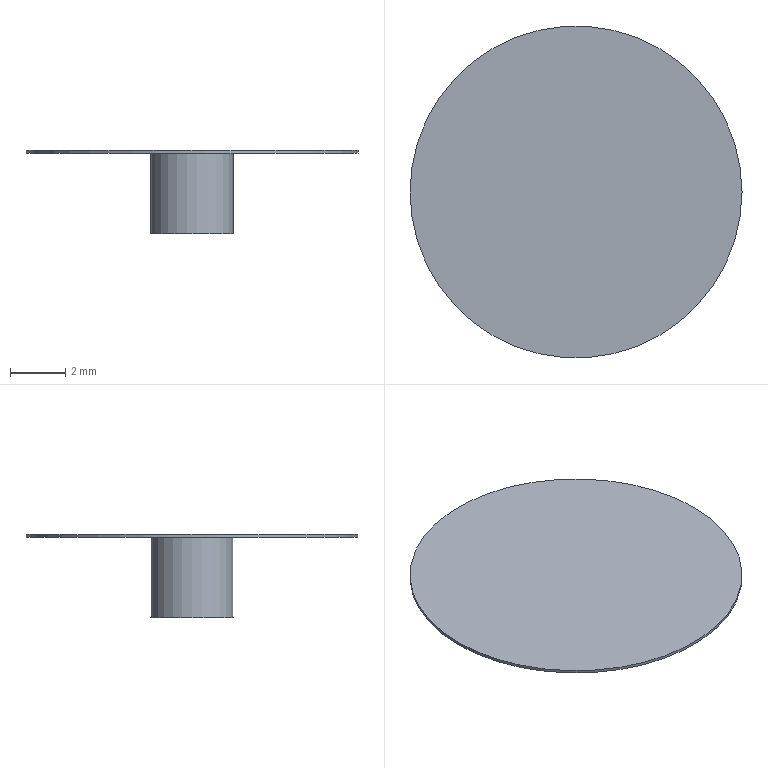Component | NX | ROBOT_ARM_FLANGE | 1 solid | 5 faces | box 12 x 12 x 3 mm | volume 32 mm3 | plane 3 | cylinder 2 | commonest cylinder face diameters 3 x1 12 x1
STEP:
#1=CARTESIAN_POINT('',(0.,0.,0.));
#2=DIRECTION('',(0.,0.,1.));
#3=DIRECTION('',(1.,0.,0.));
#4=AXIS2_PLACEMENT_3D('',#1,#2,#3);
#5=CARTESIAN_POINT('',(15.971,14.526,113.674));
#6=VERTEX_POINT('',#5);
#7=CARTESIAN_POINT('',(14.471,14.526,113.674));
#8=DIRECTION('',(0.,0.,1.));
#9=DIRECTION('',(1.,0.,0.));
#10=AXIS2_PLACEMENT_3D('',#7,#8,#9);
#11=CIRCLE('',#10,1.5);
#12=CARTESIAN_POINT('',(14.471,14.526,113.674));
#13=DIRECTION('',(0.,0.,1.));
#14=DIRECTION('',(1.,0.,0.));
#15=AXIS2_PLACEMENT_3D('',#12,#13,#14);
#16=CYLINDRICAL_SURFACE('',#15,1.5);
#17=CARTESIAN_POINT('',(0.,0.));
#18=DIRECTION('',(1.,0.));
#19=VECTOR('',#18,1.);
#20=LINE('',#17,#19);
#21=(GEOMETRIC_REPRESENTATION_CONTEXT(2)PARAMETRIC_REPRESENTATION_CONTEXT()REPRESENTATION_CONTEXT('',''));
#22=DEFINITIONAL_REPRESENTATION('',(#20),#21);
#23=PCURVE('',#16,#22);
#24=CARTESIAN_POINT('',(14.471,14.526,113.674));
#25=DIRECTION('',(0.,0.,1.));
#26=DIRECTION('',(1.,0.,0.));
#27=AXIS2_PLACEMENT_3D('',#24,#25,#26);
#28=PLANE('',#27);
#29=CARTESIAN_POINT('',(0.,0.));
#30=DIRECTION('',(1.,0.));
#31=AXIS2_PLACEMENT_2D('',#29,#30);
#32=CIRCLE('',#31,1.5);
#33=(GEOMETRIC_REPRESENTATION_CONTEXT(2)PARAMETRIC_REPRESENTATION_CONTEXT()REPRESENTATION_CONTEXT('',''));
#34=DEFINITIONAL_REPRESENTATION('',(#32),#33);
#35=PCURVE('',#28,#34);
#36=SURFACE_CURVE('',#11,(#23,#35),.PCURVE_S1.);
#37=EDGE_CURVE('',#6,#6,#36,.T.);
#38=ORIENTED_EDGE('',*,*,#37,.T.);
#39=CARTESIAN_POINT('',(15.971,14.526,116.574));
#40=VERTEX_POINT('',#39);
#41=CARTESIAN_POINT('',(15.971,14.526,113.674));
#42=CARTESIAN_POINT('',(15.971,14.526,116.574));
#43=B_SPLINE_CURVE_WITH_KNOTS('',1,(#41,#42),.UNSPECIFIED.,.F.,.F.,(2,2),(0.,2.9),.PIECEWISE_BEZIER_KNOTS.);
#44=CARTESIAN_POINT('',(6.283,0.));
#45=DIRECTION('',(0.,1.));
#46=VECTOR('',#45,1.);
#47=LINE('',#44,#46);
#48=(GEOMETRIC_REPRESENTATION_CONTEXT(2)PARAMETRIC_REPRESENTATION_CONTEXT()REPRESENTATION_CONTEXT('',''));
#49=DEFINITIONAL_REPRESENTATION('',(#47),#48);
#50=PCURVE('',#16,#49);
#51=CARTESIAN_POINT('',(0.,0.));
#52=DIRECTION('',(0.,1.));
#53=VECTOR('',#52,1.);
#54=LINE('',#51,#53);
#55=(GEOMETRIC_REPRESENTATION_CONTEXT(2)PARAMETRIC_REPRESENTATION_CONTEXT()REPRESENTATION_CONTEXT('',''));
#56=DEFINITIONAL_REPRESENTATION('',(#54),#55);
#57=PCURVE('',#16,#56);
#58=SEAM_CURVE('',#43,(#50,#57),.PCURVE_S1.);
#59=EDGE_CURVE('',#6,#40,#58,.T.);
#60=ORIENTED_EDGE('',*,*,#59,.T.);
#61=CARTESIAN_POINT('',(14.471,14.526,116.574));
#62=DIRECTION('',(0.,0.,1.));
#63=DIRECTION('',(1.,0.,0.));
#64=AXIS2_PLACEMENT_3D('',#61,#62,#63);
#65=CIRCLE('',#64,1.5);
#66=CARTESIAN_POINT('',(0.,2.9));
#67=DIRECTION('',(1.,0.));
#68=VECTOR('',#67,1.);
#69=LINE('',#66,#68);
#70=(GEOMETRIC_REPRESENTATION_CONTEXT(2)PARAMETRIC_REPRESENTATION_CONTEXT()REPRESENTATION_CONTEXT('',''));
#71=DEFINITIONAL_REPRESENTATION('',(#69),#70);
#72=PCURVE('',#16,#71);
#73=CARTESIAN_POINT('',(14.471,14.526,116.574));
#74=DIRECTION('',(0.,0.,1.));
#75=DIRECTION('',(1.,0.,0.));
#76=AXIS2_PLACEMENT_3D('',#73,#74,#75);
#77=PLANE('',#76);
#78=CARTESIAN_POINT('',(0.,0.));
#79=DIRECTION('',(1.,0.));
#80=AXIS2_PLACEMENT_2D('',#78,#79);
#81=CIRCLE('',#80,1.5);
#82=(GEOMETRIC_REPRESENTATION_CONTEXT(2)PARAMETRIC_REPRESENTATION_CONTEXT()REPRESENTATION_CONTEXT('',''));
#83=DEFINITIONAL_REPRESENTATION('',(#81),#82);
#84=PCURVE('',#77,#83);
#85=SURFACE_CURVE('',#65,(#72,#84),.PCURVE_S1.);
#86=EDGE_CURVE('',#40,#40,#85,.T.);
#87=ORIENTED_EDGE('',*,*,#86,.F.);
#88=ORIENTED_EDGE('',*,*,#59,.F.);
#89=EDGE_LOOP('',(#38,#60,#87,#88));
#90=FACE_BOUND('',#89,.T.);
#91=ADVANCED_FACE('',(#90),#16,.T.);
#92=ORIENTED_EDGE('',*,*,#37,.F.);
#93=EDGE_LOOP('',(#92));
#94=FACE_BOUND('',#93,.T.);
#95=ADVANCED_FACE('',(#94),#28,.F.);
#96=CARTESIAN_POINT('',(20.471,14.526,116.574));
#97=VERTEX_POINT('',#96);
#98=CARTESIAN_POINT('',(14.471,14.526,116.574));
#99=DIRECTION('',(0.,0.,1.));
#100=DIRECTION('',(1.,0.,0.));
#101=AXIS2_PLACEMENT_3D('',#98,#99,#100);
#102=CIRCLE('',#101,6.);
#103=CARTESIAN_POINT('',(14.471,14.526,116.574));
#104=DIRECTION('',(0.,0.,1.));
#105=DIRECTION('',(1.,0.,0.));
#106=AXIS2_PLACEMENT_3D('',#103,#104,#105);
#107=CYLINDRICAL_SURFACE('',#106,6.);
#108=CARTESIAN_POINT('',(0.,0.));
#109=DIRECTION('',(1.,0.));
#110=VECTOR('',#109,1.);
#111=LINE('',#108,#110);
#112=(GEOMETRIC_REPRESENTATION_CONTEXT(2)PARAMETRIC_REPRESENTATION_CONTEXT()REPRESENTATION_CONTEXT('',''));
#113=DEFINITIONAL_REPRESENTATION('',(#111),#112);
#114=PCURVE('',#107,#113);
#115=CARTESIAN_POINT('',(0.,0.));
#116=DIRECTION('',(1.,0.));
#117=AXIS2_PLACEMENT_2D('',#115,#116);
#118=CIRCLE('',#117,6.);
#119=(GEOMETRIC_REPRESENTATION_CONTEXT(2)PARAMETRIC_REPRESENTATION_CONTEXT()REPRESENTATION_CONTEXT('',''));
#120=DEFINITIONAL_REPRESENTATION('',(#118),#119);
#121=PCURVE('',#77,#120);
#122=SURFACE_CURVE('',#102,(#114,#121),.PCURVE_S1.);
#123=EDGE_CURVE('',#97,#97,#122,.T.);
#124=ORIENTED_EDGE('',*,*,#123,.T.);
#125=CARTESIAN_POINT('',(20.471,14.526,116.674));
#126=VERTEX_POINT('',#125);
#127=CARTESIAN_POINT('',(20.471,14.526,116.574));
#128=CARTESIAN_POINT('',(20.471,14.526,116.674));
#129=B_SPLINE_CURVE_WITH_KNOTS('',1,(#127,#128),.UNSPECIFIED.,.F.,.F.,(2,2),(0.,0.1),.PIECEWISE_BEZIER_KNOTS.);
#130=CARTESIAN_POINT('',(6.283,0.));
#131=DIRECTION('',(0.,1.));
#132=VECTOR('',#131,1.);
#133=LINE('',#130,#132);
#134=(GEOMETRIC_REPRESENTATION_CONTEXT(2)PARAMETRIC_REPRESENTATION_CONTEXT()REPRESENTATION_CONTEXT('',''));
#135=DEFINITIONAL_REPRESENTATION('',(#133),#134);
#136=PCURVE('',#107,#135);
#137=CARTESIAN_POINT('',(0.,0.));
#138=DIRECTION('',(0.,1.));
#139=VECTOR('',#138,1.);
#140=LINE('',#137,#139);
#141=(GEOMETRIC_REPRESENTATION_CONTEXT(2)PARAMETRIC_REPRESENTATION_CONTEXT()REPRESENTATION_CONTEXT('',''));
#142=DEFINITIONAL_REPRESENTATION('',(#140),#141);
#143=PCURVE('',#107,#142);
#144=SEAM_CURVE('',#129,(#136,#143),.PCURVE_S1.);
#145=EDGE_CURVE('',#97,#126,#144,.T.);
#146=ORIENTED_EDGE('',*,*,#145,.T.);
#147=CARTESIAN_POINT('',(14.471,14.526,116.674));
#148=DIRECTION('',(0.,0.,1.));
#149=DIRECTION('',(1.,0.,0.));
#150=AXIS2_PLACEMENT_3D('',#147,#148,#149);
#151=CIRCLE('',#150,6.);
#152=CARTESIAN_POINT('',(0.,0.1));
#153=DIRECTION('',(1.,0.));
#154=VECTOR('',#153,1.);
#155=LINE('',#152,#154);
#156=(GEOMETRIC_REPRESENTATION_CONTEXT(2)PARAMETRIC_REPRESENTATION_CONTEXT()REPRESENTATION_CONTEXT('',''));
#157=DEFINITIONAL_REPRESENTATION('',(#155),#156);
#158=PCURVE('',#107,#157);
#159=CARTESIAN_POINT('',(14.471,14.526,116.674));
#160=DIRECTION('',(0.,0.,1.));
#161=DIRECTION('',(1.,0.,0.));
#162=AXIS2_PLACEMENT_3D('',#159,#160,#161);
#163=PLANE('',#162);
#164=CARTESIAN_POINT('',(0.,0.));
#165=DIRECTION('',(1.,0.));
#166=AXIS2_PLACEMENT_2D('',#164,#165);
#167=CIRCLE('',#166,6.);
#168=(GEOMETRIC_REPRESENTATION_CONTEXT(2)PARAMETRIC_REPRESENTATION_CONTEXT()REPRESENTATION_CONTEXT('',''));
#169=DEFINITIONAL_REPRESENTATION('',(#167),#168);
#170=PCURVE('',#163,#169);
#171=SURFACE_CURVE('',#151,(#158,#170),.PCURVE_S1.);
#172=EDGE_CURVE('',#126,#126,#171,.T.);
#173=ORIENTED_EDGE('',*,*,#172,.F.);
#174=ORIENTED_EDGE('',*,*,#145,.F.);
#175=EDGE_LOOP('',(#124,#146,#173,#174));
#176=FACE_BOUND('',#175,.T.);
#177=ADVANCED_FACE('',(#176),#107,.T.);
#178=ORIENTED_EDGE('',*,*,#123,.F.);
#179=EDGE_LOOP('',(#178));
#180=FACE_BOUND('',#179,.T.);
#181=ORIENTED_EDGE('',*,*,#86,.T.);
#182=EDGE_LOOP('',(#181));
#183=FACE_BOUND('',#182,.T.);
#184=ADVANCED_FACE('',(#180,#183),#77,.F.);
#185=ORIENTED_EDGE('',*,*,#172,.T.);
#186=EDGE_LOOP('',(#185));
#187=FACE_BOUND('',#186,.T.);
#188=ADVANCED_FACE('',(#187),#163,.T.);
#189=CLOSED_SHELL('',(#91,#95,#177,#184,#188));
#190=MANIFOLD_SOLID_BREP('',#189);
#191=(LENGTH_UNIT()NAMED_UNIT(*)SI_UNIT(.MILLI.,.METRE.));
#192=UNCERTAINTY_MEASURE_WITH_UNIT(LENGTH_MEASURE(0.00001),#191,'','');
#193=(NAMED_UNIT(*)PLANE_ANGLE_UNIT()SI_UNIT($,.RADIAN.));
#194=(NAMED_UNIT(*)SI_UNIT($,.STERADIAN.)SOLID_ANGLE_UNIT());
#195=(GEOMETRIC_REPRESENTATION_CONTEXT(3)GLOBAL_UNCERTAINTY_ASSIGNED_CONTEXT((#192))GLOBAL_UNIT_ASSIGNED_CONTEXT((#191,#193,#194))REPRESENTATION_CONTEXT('',''));
#196=ADVANCED_BREP_SHAPE_REPRESENTATION('',(#4,#190),#195);